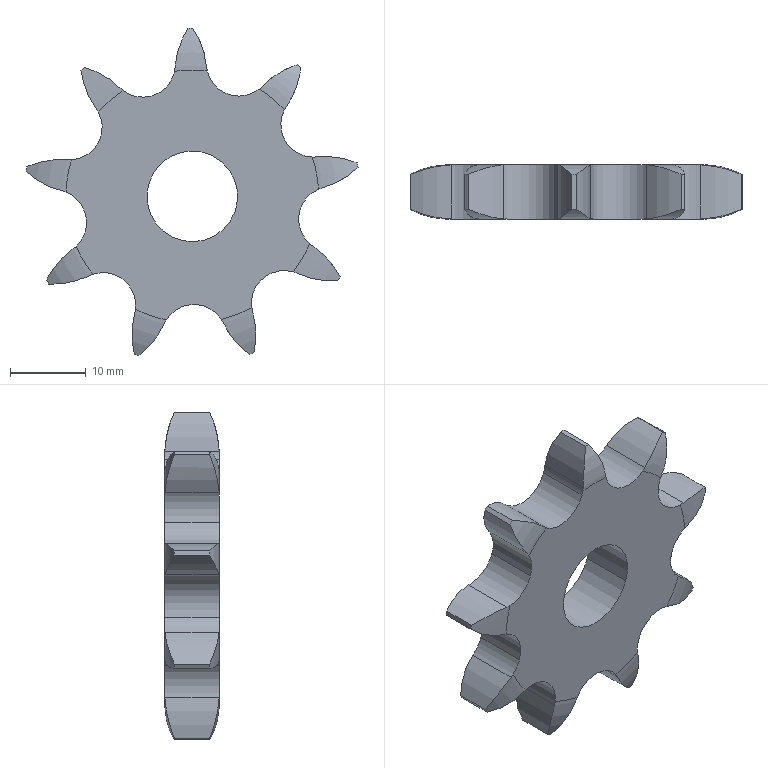Component | SolidWorks | short pitch roller chain wheel_s_iso-1 | 1 solid | 62 faces | volume 5706 mm3 | cylinder 42 | torus 18 | plane 2 | commonest cylinder face diameters 22.466 x19 8.595 x12 44.497 x9 12 x2